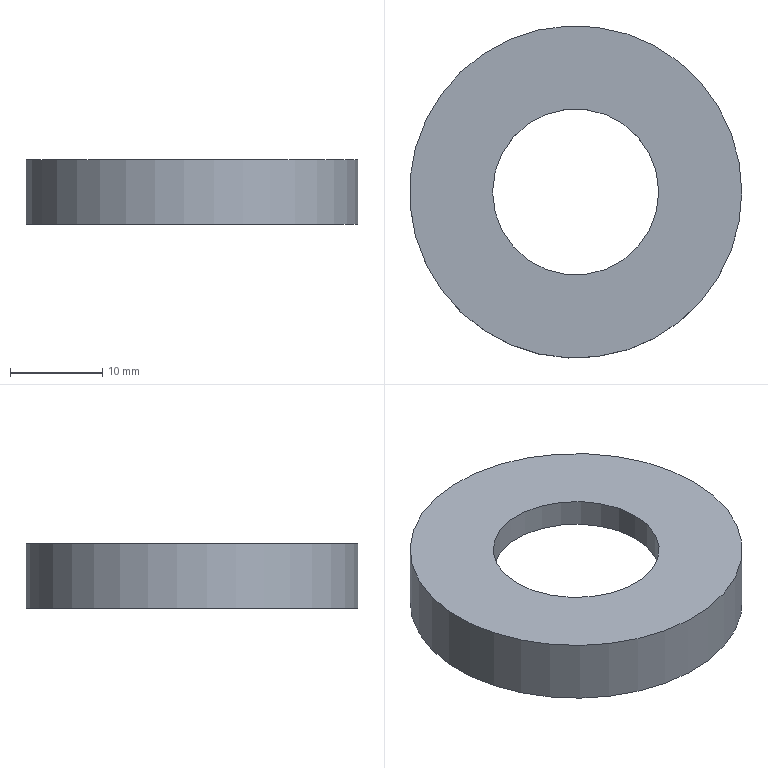Component | NX | SPHERICALWASHER | 1 solid | 5 faces | box 36 x 36 x 7 mm | volume 4088 mm3 | cylinder 2 | plane 2 | spline 1 | commonest cylinder face diameters 36 x1 18 x1
STEP:
#1=CARTESIAN_POINT('',(0.,0.,0.));
#2=DIRECTION('',(0.,0.,1.));
#3=DIRECTION('',(1.,0.,0.));
#4=AXIS2_PLACEMENT_3D('',#1,#2,#3);
#5=CARTESIAN_POINT('',(22.835,7.63,336.973));
#6=VERTEX_POINT('',#5);
#7=CARTESIAN_POINT('',(4.835,7.63,336.973));
#8=DIRECTION('',(0.,0.,-1.));
#9=DIRECTION('',(1.,0.,0.));
#10=AXIS2_PLACEMENT_3D('',#7,#8,#9);
#11=CIRCLE('',#10,18.);
#12=CARTESIAN_POINT('',(4.835,7.63,343.973));
#13=DIRECTION('',(0.,0.,-1.));
#14=DIRECTION('',(1.,0.,0.));
#15=AXIS2_PLACEMENT_3D('',#12,#13,#14);
#16=CYLINDRICAL_SURFACE('',#15,18.);
#17=CARTESIAN_POINT('',(0.,7.));
#18=DIRECTION('',(1.,0.));
#19=VECTOR('',#18,1.);
#20=LINE('',#17,#19);
#21=(GEOMETRIC_REPRESENTATION_CONTEXT(2)PARAMETRIC_REPRESENTATION_CONTEXT()REPRESENTATION_CONTEXT('',''));
#22=DEFINITIONAL_REPRESENTATION('',(#20),#21);
#23=PCURVE('',#16,#22);
#24=CARTESIAN_POINT('',(-13.165,7.63,336.973));
#25=DIRECTION('',(0.,0.,1.));
#26=DIRECTION('',(-1.,0.,0.));
#27=AXIS2_PLACEMENT_3D('',#24,#25,#26);
#28=PLANE('',#27);
#29=CARTESIAN_POINT('',(-36.,0.));
#30=CARTESIAN_POINT('',(-36.,31.177));
#31=CARTESIAN_POINT('',(-9.,15.588));
#32=CARTESIAN_POINT('',(18.,0.));
#33=CARTESIAN_POINT('',(-9.,-15.588));
#34=CARTESIAN_POINT('',(-36.,-31.177));
#35=CARTESIAN_POINT('',(-36.,0.));
#36=(BOUNDED_CURVE()B_SPLINE_CURVE(2,(#29,#30,#31,#32,#33,#34,#35),.UNSPECIFIED.,.T.,.F.)B_SPLINE_CURVE_WITH_KNOTS((1,2,2,2,2,1),(-2.094,0.,2.094,4.189,6.283,8.378),.UNSPECIFIED.)CURVE()GEOMETRIC_REPRESENTATION_ITEM()RATIONAL_B_SPLINE_CURVE((1.,0.5,1.,0.5,1.,0.5,1.))REPRESENTATION_ITEM(''));
#37=(GEOMETRIC_REPRESENTATION_CONTEXT(2)PARAMETRIC_REPRESENTATION_CONTEXT()REPRESENTATION_CONTEXT('',''));
#38=DEFINITIONAL_REPRESENTATION('',(#36),#37);
#39=PCURVE('',#28,#38);
#40=SURFACE_CURVE('',#11,(#23,#39),.PCURVE_S1.);
#41=EDGE_CURVE('',#6,#6,#40,.T.);
#42=ORIENTED_EDGE('',*,*,#41,.F.);
#43=CARTESIAN_POINT('',(22.835,7.63,343.973));
#44=VERTEX_POINT('',#43);
#45=CARTESIAN_POINT('',(22.835,7.63,343.973));
#46=CARTESIAN_POINT('',(22.835,7.63,336.973));
#47=B_SPLINE_CURVE_WITH_KNOTS('',1,(#45,#46),.UNSPECIFIED.,.F.,.F.,(2,2),(0.,7.),.PIECEWISE_BEZIER_KNOTS.);
#48=CARTESIAN_POINT('',(0.,0.));
#49=DIRECTION('',(0.,1.));
#50=VECTOR('',#49,1.);
#51=LINE('',#48,#50);
#52=(GEOMETRIC_REPRESENTATION_CONTEXT(2)PARAMETRIC_REPRESENTATION_CONTEXT()REPRESENTATION_CONTEXT('',''));
#53=DEFINITIONAL_REPRESENTATION('',(#51),#52);
#54=PCURVE('',#16,#53);
#55=CARTESIAN_POINT('',(6.283,0.));
#56=DIRECTION('',(0.,1.));
#57=VECTOR('',#56,1.);
#58=LINE('',#55,#57);
#59=(GEOMETRIC_REPRESENTATION_CONTEXT(2)PARAMETRIC_REPRESENTATION_CONTEXT()REPRESENTATION_CONTEXT('',''));
#60=DEFINITIONAL_REPRESENTATION('',(#58),#59);
#61=PCURVE('',#16,#60);
#62=SEAM_CURVE('',#47,(#54,#61),.PCURVE_S1.);
#63=EDGE_CURVE('',#44,#6,#62,.T.);
#64=ORIENTED_EDGE('',*,*,#63,.F.);
#65=CARTESIAN_POINT('',(4.835,7.63,343.973));
#66=DIRECTION('',(0.,0.,-1.));
#67=DIRECTION('',(1.,0.,0.));
#68=AXIS2_PLACEMENT_3D('',#65,#66,#67);
#69=CIRCLE('',#68,18.);
#70=CARTESIAN_POINT('',(0.,0.));
#71=DIRECTION('',(1.,0.));
#72=VECTOR('',#71,1.);
#73=LINE('',#70,#72);
#74=(GEOMETRIC_REPRESENTATION_CONTEXT(2)PARAMETRIC_REPRESENTATION_CONTEXT()REPRESENTATION_CONTEXT('',''));
#75=DEFINITIONAL_REPRESENTATION('',(#73),#74);
#76=PCURVE('',#16,#75);
#77=CARTESIAN_POINT('',(-4.165,7.63,343.973));
#78=DIRECTION('',(0.,0.,-1.));
#79=DIRECTION('',(1.,0.,0.));
#80=AXIS2_PLACEMENT_3D('',#77,#78,#79);
#81=PLANE('',#80);
#82=CARTESIAN_POINT('',(9.,0.));
#83=DIRECTION('',(1.,0.));
#84=AXIS2_PLACEMENT_2D('',#82,#83);
#85=CIRCLE('',#84,18.);
#86=(GEOMETRIC_REPRESENTATION_CONTEXT(2)PARAMETRIC_REPRESENTATION_CONTEXT()REPRESENTATION_CONTEXT('',''));
#87=DEFINITIONAL_REPRESENTATION('',(#85),#86);
#88=PCURVE('',#81,#87);
#89=SURFACE_CURVE('',#69,(#76,#88),.PCURVE_S1.);
#90=EDGE_CURVE('',#44,#44,#89,.T.);
#91=ORIENTED_EDGE('',*,*,#90,.T.);
#92=ORIENTED_EDGE('',*,*,#63,.T.);
#93=EDGE_LOOP('',(#42,#64,#91,#92));
#94=FACE_BOUND('',#93,.T.);
#95=ADVANCED_FACE('',(#94),#16,.T.);
#96=CARTESIAN_POINT('',(21.335,7.63,336.973));
#97=VERTEX_POINT('',#96);
#98=CARTESIAN_POINT('',(4.835,7.63,336.973));
#99=DIRECTION('',(0.,0.,-1.));
#100=DIRECTION('',(1.,0.,0.));
#101=AXIS2_PLACEMENT_3D('',#98,#99,#100);
#102=CIRCLE('',#101,16.5);
#103=CARTESIAN_POINT('',(-34.5,0.));
#104=CARTESIAN_POINT('',(-34.5,28.579));
#105=CARTESIAN_POINT('',(-9.75,14.289));
#106=CARTESIAN_POINT('',(15.,0.));
#107=CARTESIAN_POINT('',(-9.75,-14.289));
#108=CARTESIAN_POINT('',(-34.5,-28.579));
#109=CARTESIAN_POINT('',(-34.5,0.));
#110=(BOUNDED_CURVE()B_SPLINE_CURVE(2,(#103,#104,#105,#106,#107,#108,#109),.UNSPECIFIED.,.T.,.F.)B_SPLINE_CURVE_WITH_KNOTS((1,2,2,2,2,1),(-2.094,0.,2.094,4.189,6.283,8.378),.UNSPECIFIED.)CURVE()GEOMETRIC_REPRESENTATION_ITEM()RATIONAL_B_SPLINE_CURVE((1.,0.5,1.,0.5,1.,0.5,1.))REPRESENTATION_ITEM(''));
#111=(GEOMETRIC_REPRESENTATION_CONTEXT(2)PARAMETRIC_REPRESENTATION_CONTEXT()REPRESENTATION_CONTEXT('',''));
#112=DEFINITIONAL_REPRESENTATION('',(#110),#111);
#113=PCURVE('',#28,#112);
#114=CARTESIAN_POINT('',(13.835,7.63,340.973));
#115=CARTESIAN_POINT('',(13.835,-10.37,340.973));
#116=CARTESIAN_POINT('',(-4.165,-10.37,340.973));
#117=CARTESIAN_POINT('',(-4.165,7.63,340.973));
#118=CARTESIAN_POINT('',(-4.165,25.63,340.973));
#119=CARTESIAN_POINT('',(13.835,25.63,340.973));
#120=CARTESIAN_POINT('',(13.835,7.63,340.973));
#121=CARTESIAN_POINT('',(16.561,7.63,340.094));
#122=CARTESIAN_POINT('',(16.561,-15.82,340.094));
#123=CARTESIAN_POINT('',(-6.89,-15.82,340.094));
#124=CARTESIAN_POINT('',(-6.89,7.63,340.094));
#125=CARTESIAN_POINT('',(-6.89,31.081,340.094));
#126=CARTESIAN_POINT('',(16.561,31.081,340.094));
#127=CARTESIAN_POINT('',(16.561,7.63,340.094));
#128=CARTESIAN_POINT('',(19.087,7.63,338.746));
#129=CARTESIAN_POINT('',(19.087,-20.873,338.746));
#130=CARTESIAN_POINT('',(-9.417,-20.873,338.746));
#131=CARTESIAN_POINT('',(-9.417,7.63,338.746));
#132=CARTESIAN_POINT('',(-9.417,36.134,338.746));
#133=CARTESIAN_POINT('',(19.087,36.134,338.746));
#134=CARTESIAN_POINT('',(19.087,7.63,338.746));
#135=CARTESIAN_POINT('',(21.335,7.63,336.973));
#136=CARTESIAN_POINT('',(21.335,-25.37,336.973));
#137=CARTESIAN_POINT('',(-11.665,-25.37,336.973));
#138=CARTESIAN_POINT('',(-11.665,7.63,336.973));
#139=CARTESIAN_POINT('',(-11.665,40.63,336.973));
#140=CARTESIAN_POINT('',(21.335,40.63,336.973));
#141=CARTESIAN_POINT('',(21.335,7.63,336.973));
#142=(BOUNDED_SURFACE()B_SPLINE_SURFACE(3,3,((#114,#115,#116,#117,#118,#119,#120),(#121,#122,#123,#124,#125,#126,#127),(#128,#129,#130,#131,#132,#133,#134),(#135,#136,#137,#138,#139,#140,#141)),.UNSPECIFIED.,.F.,.T.,.F.)B_SPLINE_SURFACE_WITH_KNOTS((4,4),(1,3,3,3,1),(0.,1.),(-0.5,0.,0.5,1.,1.5),.UNSPECIFIED.)GEOMETRIC_REPRESENTATION_ITEM()RATIONAL_B_SPLINE_SURFACE(((1.,0.3333,0.3333,1.,0.3333,0.3333,1.),(0.9895,0.3298,0.3298,0.9895,0.3298,0.3298,0.9895),(0.9895,0.3298,0.3298,0.9895,0.3298,0.3298,0.9895),(1.,0.3333,0.3333,1.,0.3333,0.3333,1.)))REPRESENTATION_ITEM('')SURFACE());
#143=CARTESIAN_POINT('',(1.,0.));
#144=CARTESIAN_POINT('',(1.,0.02352));
#145=CARTESIAN_POINT('',(1.,0.06491));
#146=CARTESIAN_POINT('',(1.,0.1146));
#147=CARTESIAN_POINT('',(1.,0.1575));
#148=CARTESIAN_POINT('',(1.,0.196));
#149=CARTESIAN_POINT('',(1.,0.2322));
#150=CARTESIAN_POINT('',(1.,0.2678));
#151=CARTESIAN_POINT('',(1.,0.304));
#152=CARTESIAN_POINT('',(1.,0.3425));
#153=CARTESIAN_POINT('',(1.,0.3856));
#154=CARTESIAN_POINT('',(1.,0.4343));
#155=CARTESIAN_POINT('',(1.,0.5));
#156=CARTESIAN_POINT('',(1.,0.5657));
#157=CARTESIAN_POINT('',(1.,0.6144));
#158=CARTESIAN_POINT('',(1.,0.6575));
#159=CARTESIAN_POINT('',(1.,0.696));
#160=CARTESIAN_POINT('',(1.,0.7322));
#161=CARTESIAN_POINT('',(1.,0.7678));
#162=CARTESIAN_POINT('',(1.,0.804));
#163=CARTESIAN_POINT('',(1.,0.8425));
#164=CARTESIAN_POINT('',(1.,0.8854));
#165=CARTESIAN_POINT('',(1.,0.9351));
#166=CARTESIAN_POINT('',(1.,0.9765));
#167=CARTESIAN_POINT('',(1.,1.));
#168=B_SPLINE_CURVE_WITH_KNOTS('',3,(#143,#144,#145,#146,#147,#148,#149,#150,#151,#152,#153,#154,#155,#156,#157,#158,#159,#160,#161,#162,#163,#164,#165,#166,#167),.UNSPECIFIED.,.F.,.F.,(4,1,1,1,1,1,1,1,1,1,1,1,1,1,1,1,1,1,1,1,1,1,4),(0.,0.2856,0.5712,0.8568,1.142,1.428,1.714,1.999,2.285,2.57,2.856,3.142,3.427,3.713,3.998,4.284,4.57,4.855,5.141,5.426,5.712,5.998,6.283),.QUASI_UNIFORM_KNOTS.);
#169=(GEOMETRIC_REPRESENTATION_CONTEXT(2)PARAMETRIC_REPRESENTATION_CONTEXT()REPRESENTATION_CONTEXT('',''));
#170=DEFINITIONAL_REPRESENTATION('',(#168),#169);
#171=PCURVE('',#142,#170);
#172=SURFACE_CURVE('',#102,(#113,#171),.PCURVE_S1.);
#173=EDGE_CURVE('',#97,#97,#172,.T.);
#174=ORIENTED_EDGE('',*,*,#173,.F.);
#175=EDGE_LOOP('',(#174));
#176=FACE_BOUND('',#175,.T.);
#177=ORIENTED_EDGE('',*,*,#41,.T.);
#178=EDGE_LOOP('',(#177));
#179=FACE_BOUND('',#178,.T.);
#180=ADVANCED_FACE('',(#176,#179),#28,.F.);
#181=CARTESIAN_POINT('',(13.835,7.63,340.973));
#182=VERTEX_POINT('',#181);
#183=CARTESIAN_POINT('',(4.835,7.63,340.973));
#184=DIRECTION('',(0.,0.,-1.));
#185=DIRECTION('',(1.,0.,0.));
#186=AXIS2_PLACEMENT_3D('',#183,#184,#185);
#187=CIRCLE('',#186,9.);
#188=CARTESIAN_POINT('',(0.,0.));
#189=CARTESIAN_POINT('',(0.,0.02352));
#190=CARTESIAN_POINT('',(0.,0.06491));
#191=CARTESIAN_POINT('',(0.,0.1146));
#192=CARTESIAN_POINT('',(0.,0.1575));
#193=CARTESIAN_POINT('',(0.,0.196));
#194=CARTESIAN_POINT('',(0.,0.2322));
#195=CARTESIAN_POINT('',(0.,0.2678));
#196=CARTESIAN_POINT('',(0.,0.304));
#197=CARTESIAN_POINT('',(0.,0.3425));
#198=CARTESIAN_POINT('',(0.,0.3856));
#199=CARTESIAN_POINT('',(0.,0.4343));
#200=CARTESIAN_POINT('',(0.,0.5));
#201=CARTESIAN_POINT('',(0.,0.5657));
#202=CARTESIAN_POINT('',(0.,0.6144));
#203=CARTESIAN_POINT('',(0.,0.6575));
#204=CARTESIAN_POINT('',(0.,0.696));
#205=CARTESIAN_POINT('',(0.,0.7322));
#206=CARTESIAN_POINT('',(0.,0.7678));
#207=CARTESIAN_POINT('',(0.,0.804));
#208=CARTESIAN_POINT('',(0.,0.8425));
#209=CARTESIAN_POINT('',(0.,0.8854));
#210=CARTESIAN_POINT('',(0.,0.9351));
#211=CARTESIAN_POINT('',(0.,0.9765));
#212=CARTESIAN_POINT('',(0.,1.));
#213=B_SPLINE_CURVE_WITH_KNOTS('',3,(#188,#189,#190,#191,#192,#193,#194,#195,#196,#197,#198,#199,#200,#201,#202,#203,#204,#205,#206,#207,#208,#209,#210,#211,#212),.UNSPECIFIED.,.F.,.F.,(4,1,1,1,1,1,1,1,1,1,1,1,1,1,1,1,1,1,1,1,1,1,4),(0.,0.2856,0.5712,0.8568,1.142,1.428,1.714,1.999,2.285,2.57,2.856,3.142,3.427,3.713,3.998,4.284,4.57,4.855,5.141,5.426,5.712,5.998,6.283),.QUASI_UNIFORM_KNOTS.);
#214=(GEOMETRIC_REPRESENTATION_CONTEXT(2)PARAMETRIC_REPRESENTATION_CONTEXT()REPRESENTATION_CONTEXT('',''));
#215=DEFINITIONAL_REPRESENTATION('',(#213),#214);
#216=PCURVE('',#142,#215);
#217=CARTESIAN_POINT('',(4.835,7.63,343.973));
#218=DIRECTION('',(0.,0.,-1.));
#219=DIRECTION('',(1.,0.,0.));
#220=AXIS2_PLACEMENT_3D('',#217,#218,#219);
#221=CYLINDRICAL_SURFACE('',#220,9.);
#222=CARTESIAN_POINT('',(0.,3.));
#223=DIRECTION('',(1.,0.));
#224=VECTOR('',#223,1.);
#225=LINE('',#222,#224);
#226=(GEOMETRIC_REPRESENTATION_CONTEXT(2)PARAMETRIC_REPRESENTATION_CONTEXT()REPRESENTATION_CONTEXT('',''));
#227=DEFINITIONAL_REPRESENTATION('',(#225),#226);
#228=PCURVE('',#221,#227);
#229=SURFACE_CURVE('',#187,(#216,#228),.PCURVE_S1.);
#230=EDGE_CURVE('',#182,#182,#229,.T.);
#231=ORIENTED_EDGE('',*,*,#230,.F.);
#232=CARTESIAN_POINT('',(13.835,7.63,340.973));
#233=CARTESIAN_POINT('',(16.561,7.63,340.094));
#234=CARTESIAN_POINT('',(19.087,7.63,338.746));
#235=CARTESIAN_POINT('',(21.335,7.63,336.973));
#236=(BOUNDED_CURVE()B_SPLINE_CURVE(3,(#232,#233,#234,#235),.UNSPECIFIED.,.F.,.F.)B_SPLINE_CURVE_WITH_KNOTS((4,4),(0.,1.),.PIECEWISE_BEZIER_KNOTS.)CURVE()GEOMETRIC_REPRESENTATION_ITEM()RATIONAL_B_SPLINE_CURVE((1.,0.9895,0.9895,1.))REPRESENTATION_ITEM(''));
#237=CARTESIAN_POINT('',(0.,0.));
#238=DIRECTION('',(1.,0.));
#239=VECTOR('',#238,1.);
#240=LINE('',#237,#239);
#241=(GEOMETRIC_REPRESENTATION_CONTEXT(2)PARAMETRIC_REPRESENTATION_CONTEXT()REPRESENTATION_CONTEXT('',''));
#242=DEFINITIONAL_REPRESENTATION('',(#240),#241);
#243=PCURVE('',#142,#242);
#244=CARTESIAN_POINT('',(0.,1.));
#245=DIRECTION('',(1.,0.));
#246=VECTOR('',#245,1.);
#247=LINE('',#244,#246);
#248=(GEOMETRIC_REPRESENTATION_CONTEXT(2)PARAMETRIC_REPRESENTATION_CONTEXT()REPRESENTATION_CONTEXT('',''));
#249=DEFINITIONAL_REPRESENTATION('',(#247),#248);
#250=PCURVE('',#142,#249);
#251=SEAM_CURVE('',#236,(#243,#250),.PCURVE_S1.);
#252=EDGE_CURVE('',#182,#97,#251,.T.);
#253=ORIENTED_EDGE('',*,*,#252,.T.);
#254=ORIENTED_EDGE('',*,*,#173,.T.);
#255=ORIENTED_EDGE('',*,*,#252,.F.);
#256=EDGE_LOOP('',(#231,#253,#254,#255));
#257=FACE_BOUND('',#256,.T.);
#258=ADVANCED_FACE('',(#257),#142,.T.);
#259=CARTESIAN_POINT('',(13.835,7.63,343.973));
#260=VERTEX_POINT('',#259);
#261=CARTESIAN_POINT('',(4.835,7.63,343.973));
#262=DIRECTION('',(0.,0.,-1.));
#263=DIRECTION('',(1.,0.,0.));
#264=AXIS2_PLACEMENT_3D('',#261,#262,#263);
#265=CIRCLE('',#264,9.);
#266=CARTESIAN_POINT('',(0.,0.));
#267=DIRECTION('',(1.,0.));
#268=VECTOR('',#267,1.);
#269=LINE('',#266,#268);
#270=(GEOMETRIC_REPRESENTATION_CONTEXT(2)PARAMETRIC_REPRESENTATION_CONTEXT()REPRESENTATION_CONTEXT('',''));
#271=DEFINITIONAL_REPRESENTATION('',(#269),#270);
#272=PCURVE('',#221,#271);
#273=CARTESIAN_POINT('',(9.,0.));
#274=DIRECTION('',(1.,0.));
#275=AXIS2_PLACEMENT_2D('',#273,#274);
#276=CIRCLE('',#275,9.);
#277=(GEOMETRIC_REPRESENTATION_CONTEXT(2)PARAMETRIC_REPRESENTATION_CONTEXT()REPRESENTATION_CONTEXT('',''));
#278=DEFINITIONAL_REPRESENTATION('',(#276),#277);
#279=PCURVE('',#81,#278);
#280=SURFACE_CURVE('',#265,(#272,#279),.PCURVE_S1.);
#281=EDGE_CURVE('',#260,#260,#280,.T.);
#282=ORIENTED_EDGE('',*,*,#281,.T.);
#283=CARTESIAN_POINT('',(13.835,7.63,343.973));
#284=CARTESIAN_POINT('',(13.835,7.63,340.973));
#285=B_SPLINE_CURVE_WITH_KNOTS('',1,(#283,#284),.UNSPECIFIED.,.F.,.F.,(2,2),(0.,3.),.PIECEWISE_BEZIER_KNOTS.);
#286=CARTESIAN_POINT('',(6.283,0.));
#287=DIRECTION('',(0.,1.));
#288=VECTOR('',#287,1.);
#289=LINE('',#286,#288);
#290=(GEOMETRIC_REPRESENTATION_CONTEXT(2)PARAMETRIC_REPRESENTATION_CONTEXT()REPRESENTATION_CONTEXT('',''));
#291=DEFINITIONAL_REPRESENTATION('',(#289),#290);
#292=PCURVE('',#221,#291);
#293=CARTESIAN_POINT('',(0.,0.));
#294=DIRECTION('',(0.,1.));
#295=VECTOR('',#294,1.);
#296=LINE('',#293,#295);
#297=(GEOMETRIC_REPRESENTATION_CONTEXT(2)PARAMETRIC_REPRESENTATION_CONTEXT()REPRESENTATION_CONTEXT('',''));
#298=DEFINITIONAL_REPRESENTATION('',(#296),#297);
#299=PCURVE('',#221,#298);
#300=SEAM_CURVE('',#285,(#292,#299),.PCURVE_S1.);
#301=EDGE_CURVE('',#260,#182,#300,.T.);
#302=ORIENTED_EDGE('',*,*,#301,.T.);
#303=ORIENTED_EDGE('',*,*,#230,.F.);
#304=ORIENTED_EDGE('',*,*,#301,.F.);
#305=EDGE_LOOP('',(#282,#302,#303,#304));
#306=FACE_BOUND('',#305,.F.);
#307=ADVANCED_FACE('',(#306),#221,.F.);
#308=ORIENTED_EDGE('',*,*,#90,.F.);
#309=EDGE_LOOP('',(#308));
#310=FACE_BOUND('',#309,.T.);
#311=ORIENTED_EDGE('',*,*,#281,.T.);
#312=EDGE_LOOP('',(#311));
#313=FACE_BOUND('',#312,.T.);
#314=ADVANCED_FACE('',(#310,#313),#81,.F.);
#315=CLOSED_SHELL('',(#95,#180,#258,#307,#314));
#316=MANIFOLD_SOLID_BREP('',#315);
#317=(LENGTH_UNIT()NAMED_UNIT(*)SI_UNIT(.MILLI.,.METRE.));
#318=UNCERTAINTY_MEASURE_WITH_UNIT(LENGTH_MEASURE(0.00001),#317,'','');
#319=(NAMED_UNIT(*)PLANE_ANGLE_UNIT()SI_UNIT($,.RADIAN.));
#320=(NAMED_UNIT(*)SI_UNIT($,.STERADIAN.)SOLID_ANGLE_UNIT());
#321=(GEOMETRIC_REPRESENTATION_CONTEXT(3)GLOBAL_UNCERTAINTY_ASSIGNED_CONTEXT((#318))GLOBAL_UNIT_ASSIGNED_CONTEXT((#317,#319,#320))REPRESENTATION_CONTEXT('',''));
#322=ADVANCED_BREP_SHAPE_REPRESENTATION('',(#4,#316),#321);